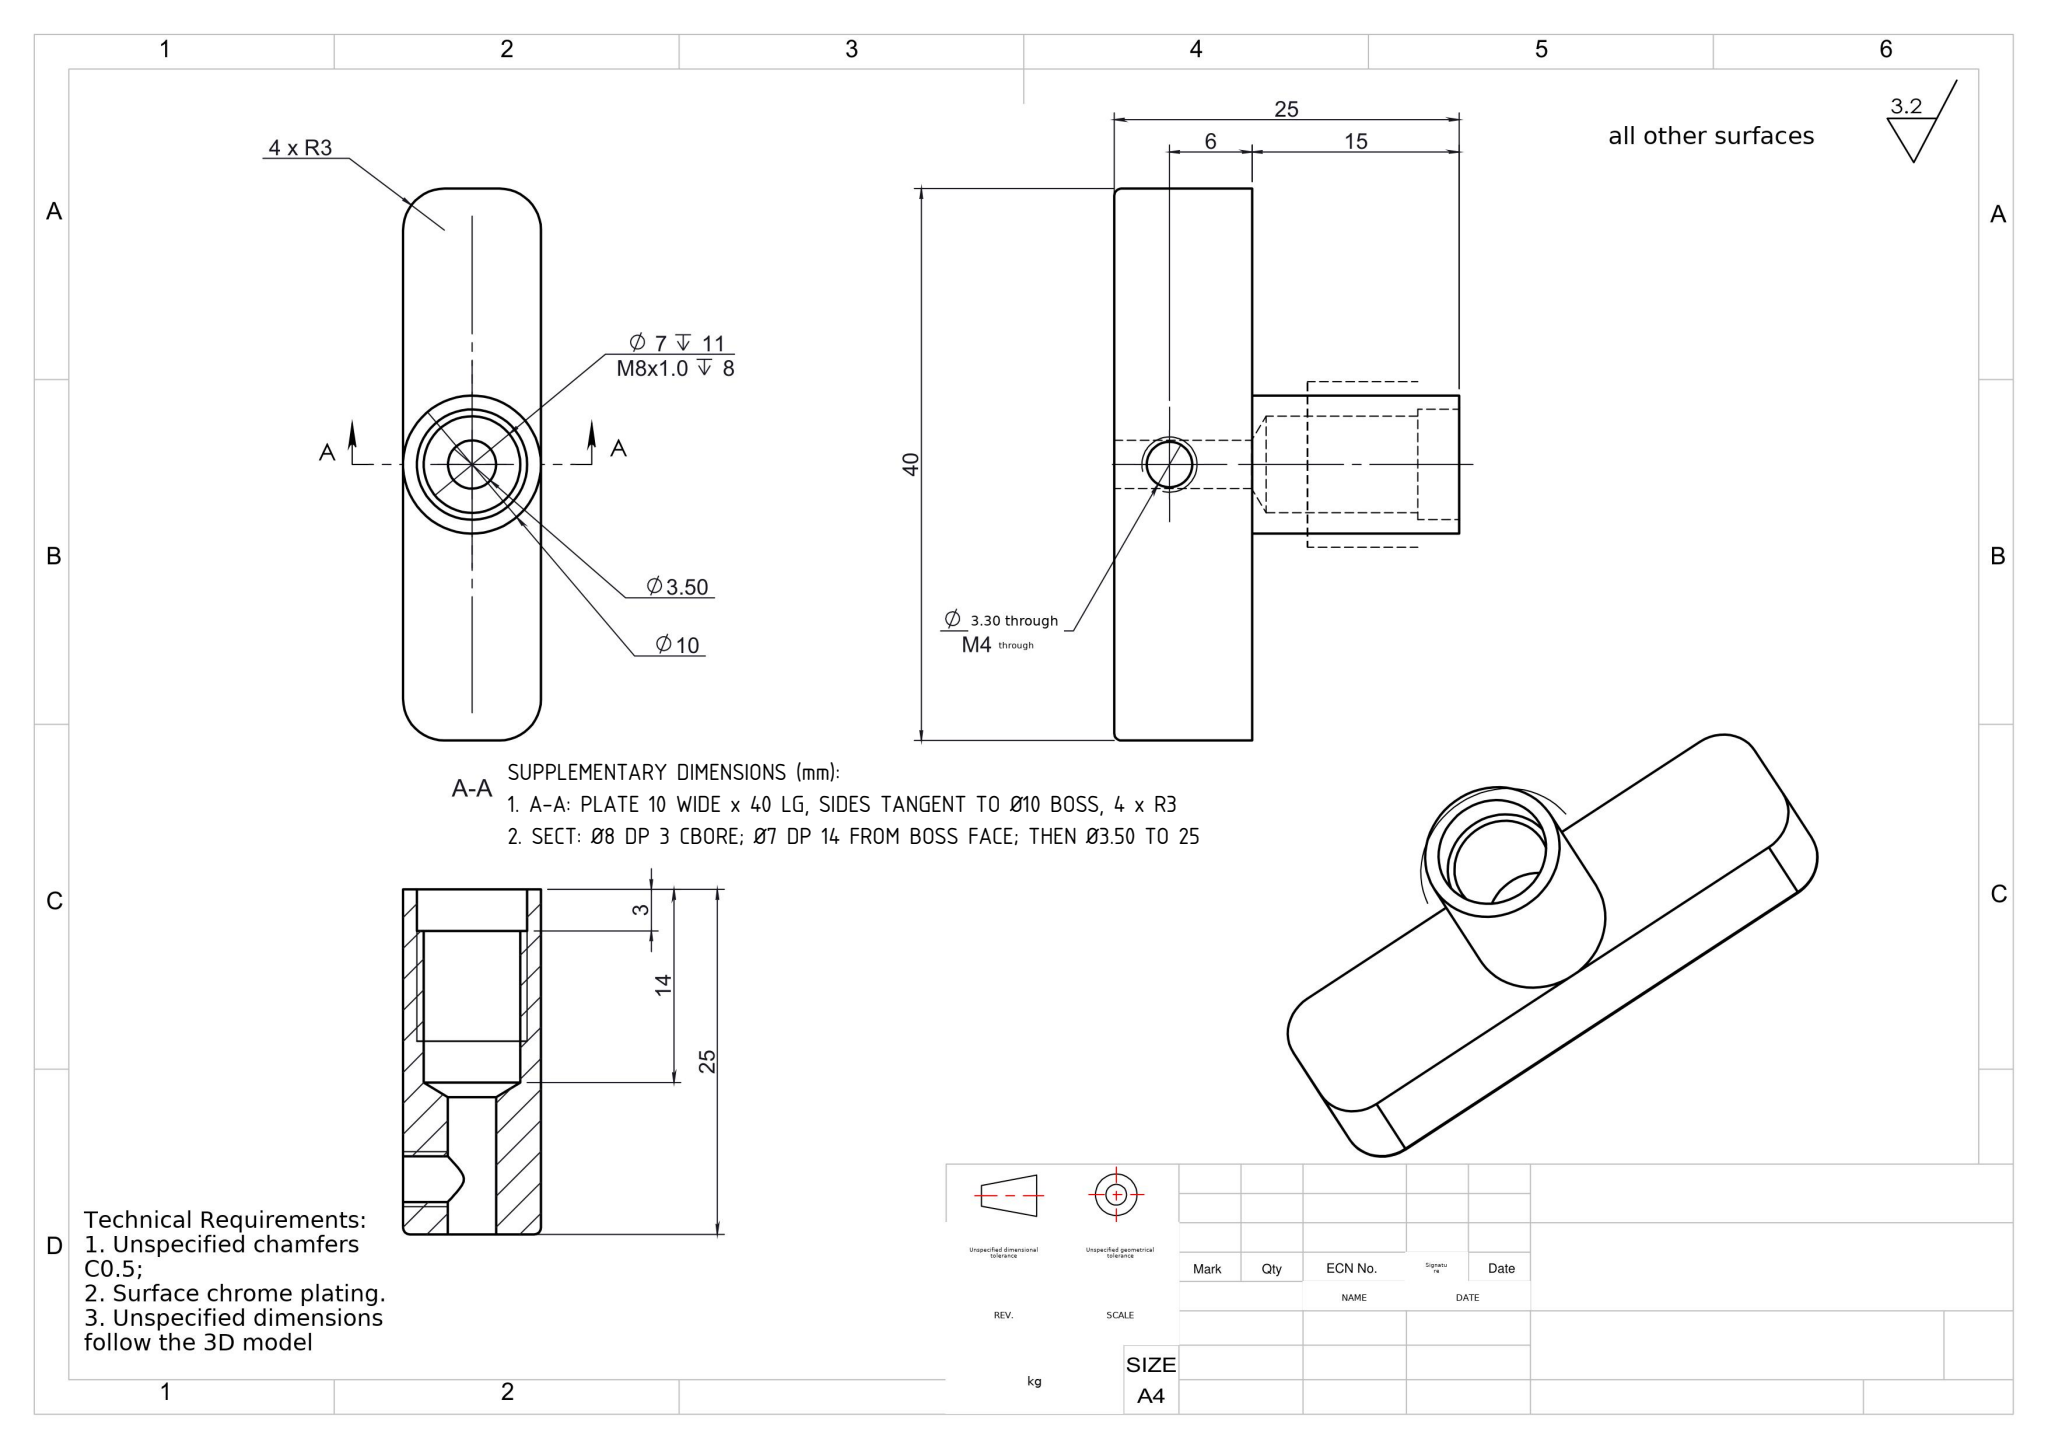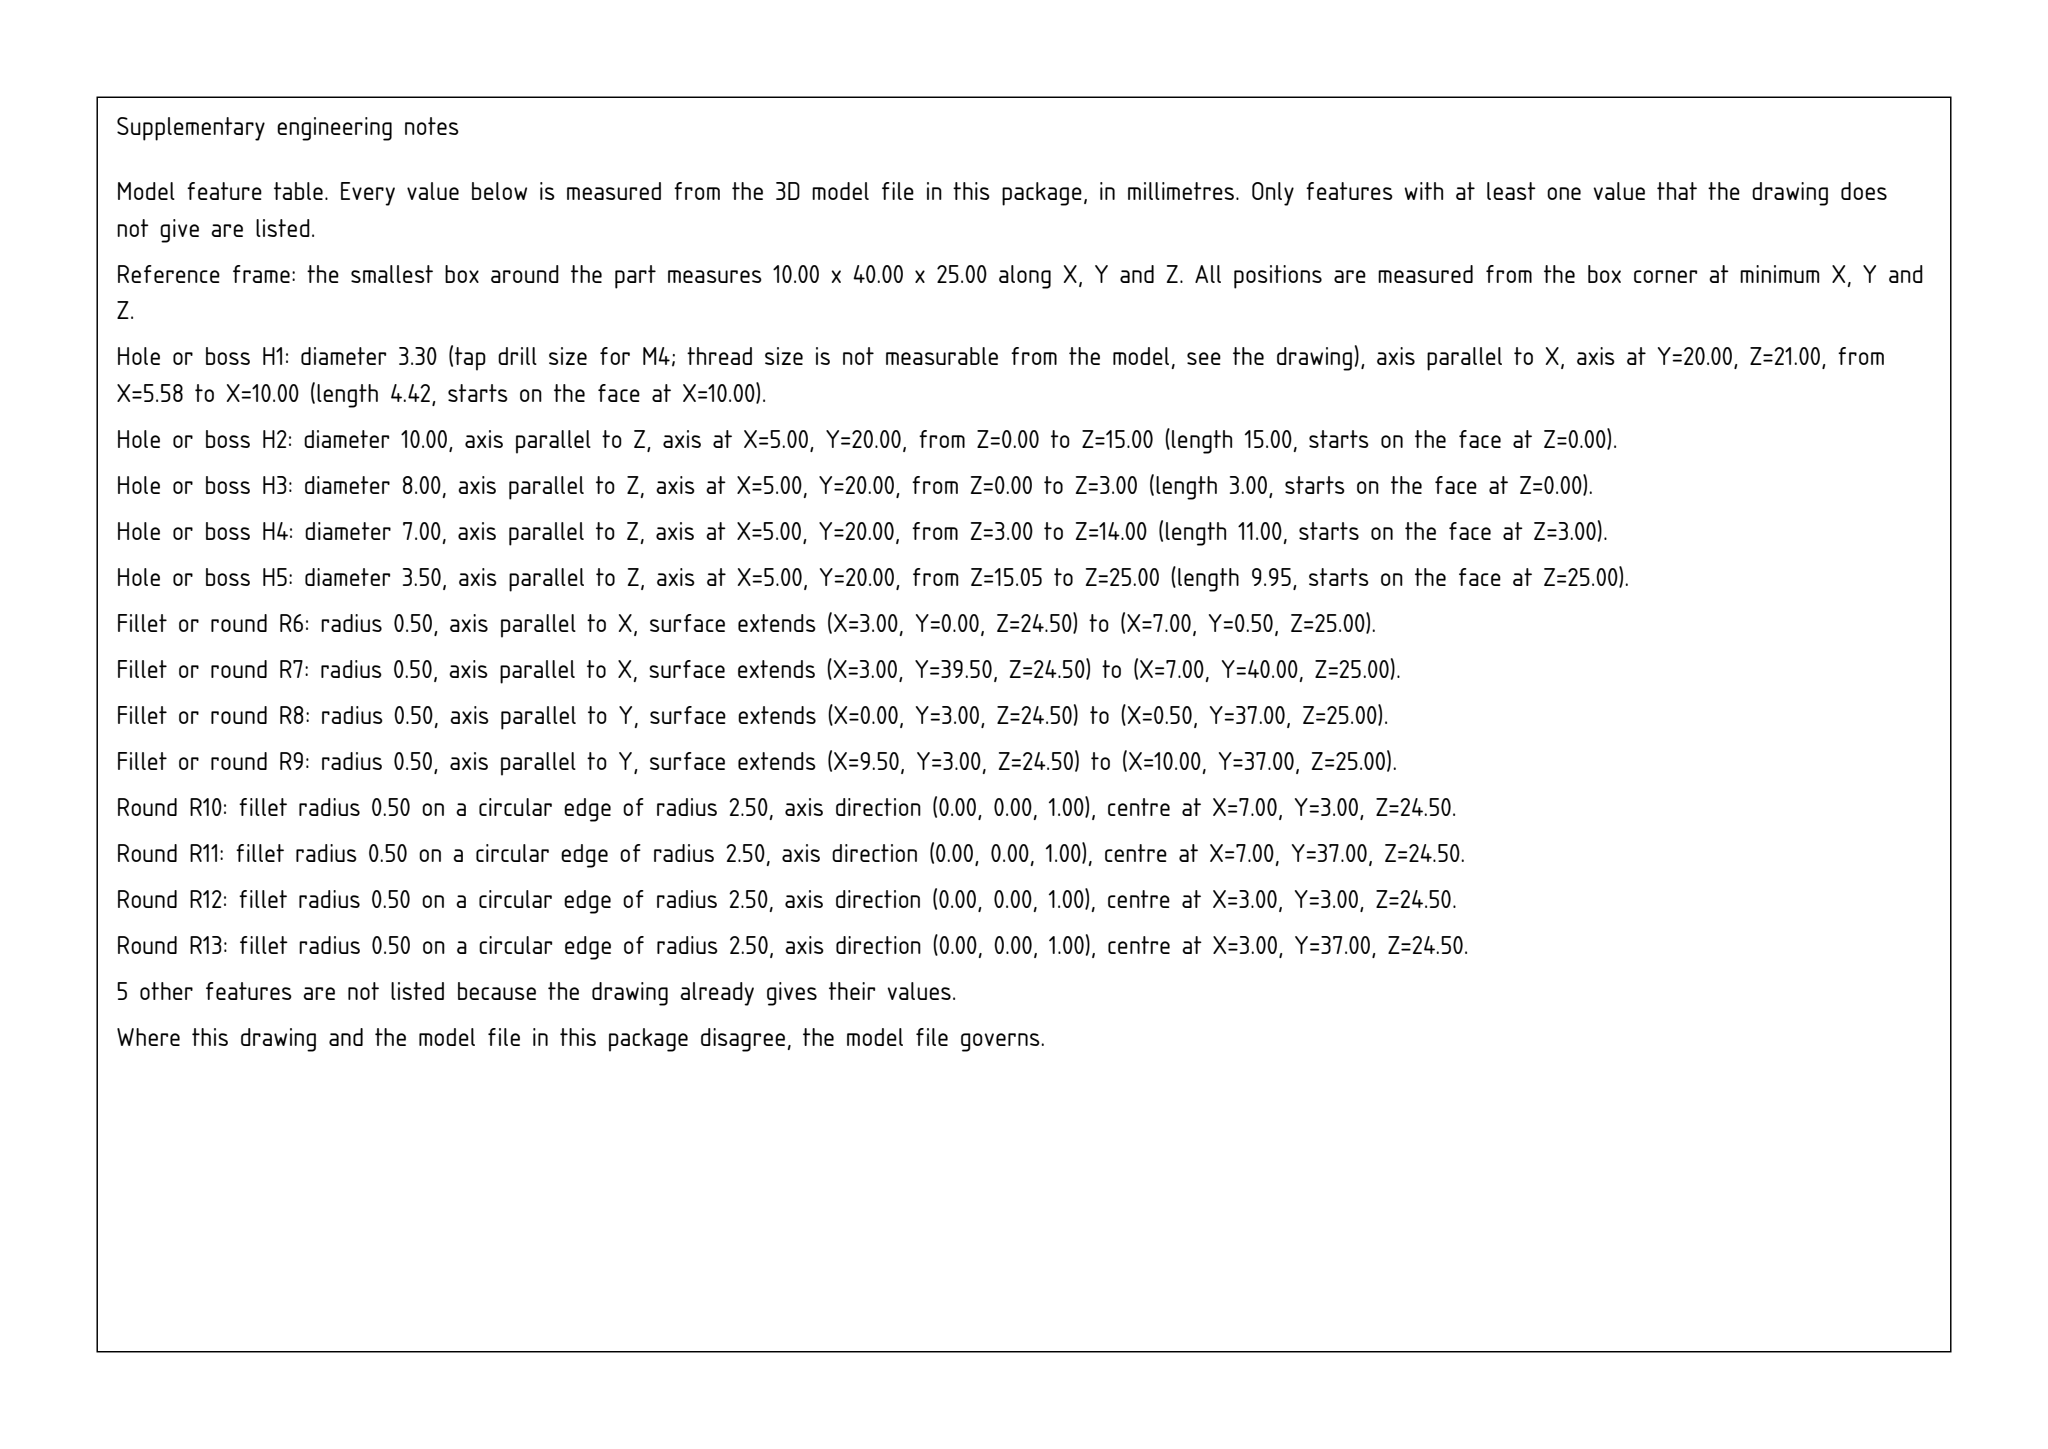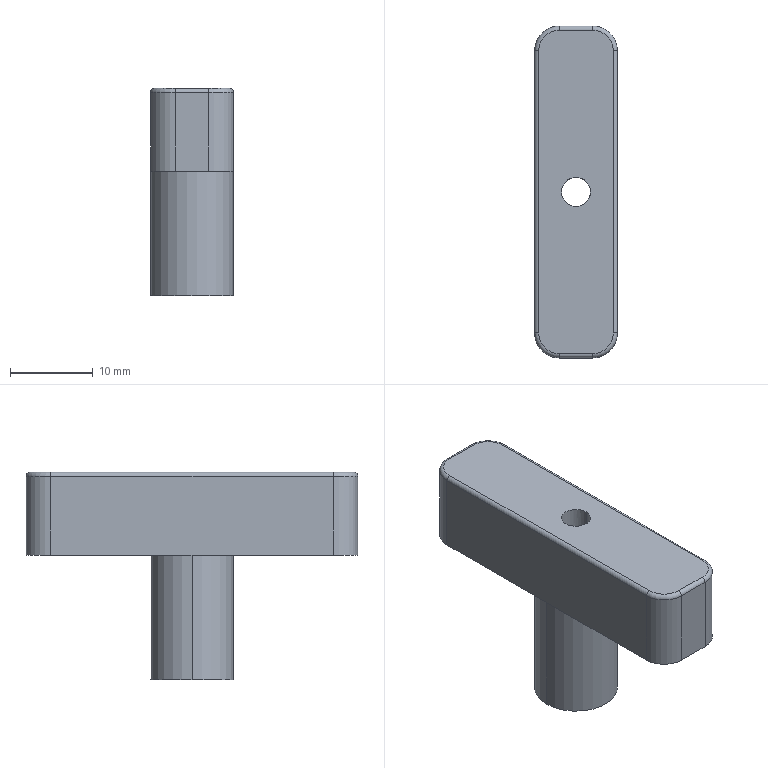Part | SolidWorks | mm | 1 solid | 33 faces | box 10 x 40 x 25 mm | volume 4373 mm3 | cylinder 18 | plane 9 | torus 4 | cone 2 | commonest cylinder face diameters 6 x4 1 x4 3.3 x2 7 x2 8 x2 10 x2 3.5 x2
build123d program:
from build123d import *

# Parameters (mm, degrees)
SKETCH1_W                 = 10
SKETCH1_H                 = 40
BOSS_EXTRUDE1_DEPTH       = 10
SKETCH2_R                 = 5
BOSS_EXTRUDE2_DEPTH       = 15
SKETCH3_R                 = 1.75
CUT_EXTRUDE1_DEPTH        = 33.404
SKETCH4_R                 = 4
CUT_EXTRUDE2_DEPTH        = 3
M8X1_0_TAPPED_HOLE1_D     = 7
M8X1_0_TAPPED_HOLE1_DEPTH = 11
M8X1_0_TAPPED_HOLE1_TIP   = 2.103
M4_TAPPED_HOLE1_REACH     = 29.299
M4_TAPPED_HOLE1_BORE_R    = 1.65
FILLET1_R                 = 3
FILLET2_R                 = 0.5


with BuildPart() as part:
    # Sketch1 → Boss-Extrude1 (new body)
    with BuildSketch(Plane.XY):
        Rectangle(SKETCH1_W, SKETCH1_H)
    extrude(amount=BOSS_EXTRUDE1_DEPTH)

    # Sketch2 → Boss-Extrude2 (add)
    with BuildSketch(Plane(origin=(0, 0, 0), x_dir=(-1, 0, 0), z_dir=(0, 0, -1))):
        Circle(SKETCH2_R)
    extrude(amount=BOSS_EXTRUDE2_DEPTH)

    # Sketch3 → Cut-Extrude1 (cut, through all)
    with BuildSketch(Plane(origin=(0, 0, -15), x_dir=(-1, 0, 0), z_dir=(0, 0, -1))):
        Circle(SKETCH3_R)
    extrude(amount=-CUT_EXTRUDE1_DEPTH, mode=Mode.SUBTRACT)

    # Sketch4 → Cut-Extrude2 (cut)
    with BuildSketch(Plane(origin=(0, 0, -15), x_dir=(-1, 0, 0), z_dir=(0, 0, -1))):
        Circle(SKETCH4_R)
    extrude(amount=-CUT_EXTRUDE2_DEPTH, mode=Mode.SUBTRACT)

    # M8x1.0 Tapped Hole1
    with Locations(Plane(origin=(0, 0, -12), x_dir=(-1, 0, 0), z_dir=(0, 0, -1))):
        with Locations((0, 0)):
            Hole(M8X1_0_TAPPED_HOLE1_D / 2, depth=M8X1_0_TAPPED_HOLE1_DEPTH)
            with Locations((0, 0, -(M8X1_0_TAPPED_HOLE1_DEPTH + M8X1_0_TAPPED_HOLE1_TIP / 2))):  # 118° drill point
                Cone(0, M8X1_0_TAPPED_HOLE1_D / 2, M8X1_0_TAPPED_HOLE1_TIP, mode=Mode.SUBTRACT)

    # M4 Tapped Hole1 bore → M4 Tapped Hole1 (cut, up to next)
    with BuildSketch(Plane(origin=(5, -0.5, 0), x_dir=(0, -1, 0), z_dir=(1, 0, 0)), mode=Mode.PRIVATE) as m4_tapped_hole1_sk1:
        with Locations((-0.5, -6)):
            Circle(M4_TAPPED_HOLE1_BORE_R)
    m4_tapped_hole1_tool1 = extrude(m4_tapped_hole1_sk1.sketch, amount=-M4_TAPPED_HOLE1_REACH, mode=Mode.PRIVATE) & part.part
    add(m4_tapped_hole1_tool1.solids().sort_by_distance((5, 0, 6))[0], mode=Mode.SUBTRACT)

    # Fillet1
    fillet1_edges = [part.edges().sort_by_distance(p)[0] for p in [
        (-5, 20, 5),
        (5, 20, 5),
        (5, -20, 5),
        (-5, -20, 5),
    ]]
    fillet(fillet1_edges, radius=FILLET1_R)

    # Fillet2
    fillet2_edges = [part.edges().sort_by_distance(p)[0] for p in [
        (0, -20, 10),
        (-5, 0, 10),
        (5, 0, 10),
        (0, 20, 10),
        (4.121, 19.121, 10),
        (-4.121, 19.121, 10),
        (4.121, -19.121, 10),
        (-4.121, -19.121, 10),
    ]]
    fillet(fillet2_edges, radius=FILLET2_R)


solid = part.part